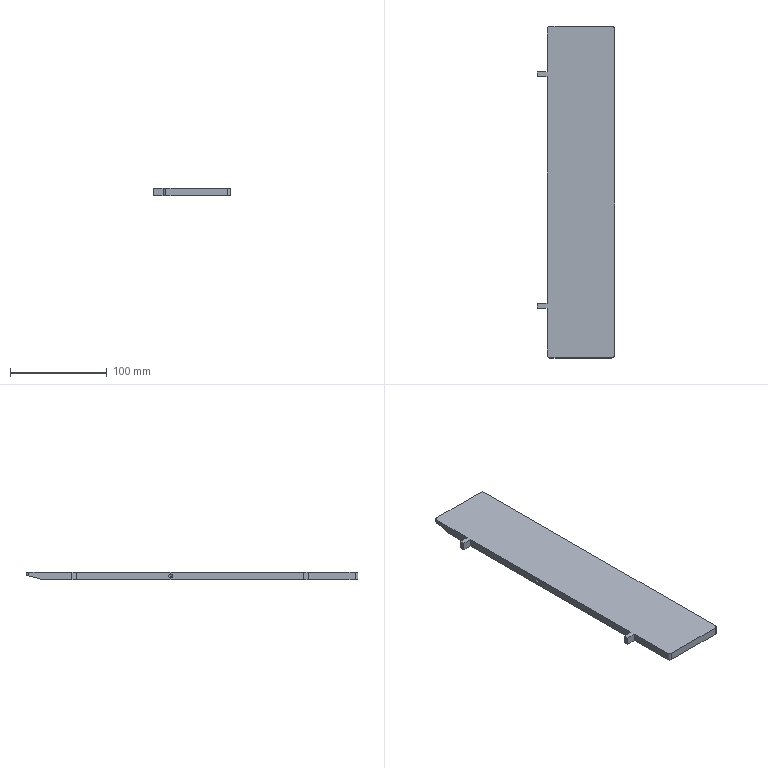Component | SolidWorks | SecondGenerationFour-sidedLabelingFeedingRearBaffle-1 | 1 solid | 23 faces | box 80 x 344 x 8 mm | volume 189871 mm3 | plane 15 | cylinder 6 | cone 2 | commonest cylinder face diameters 6 x4 4.2 x2
build123d program:
from build123d import *

# Parameters (mm, degrees)
SKETCH1_W             = 8
SKETCH1_H             = 345
BOSS_EXTRUDE1_DEPTH   = 70
M5_TAPPED_HOLE1_D     = 4.2
M5_TAPPED_HOLE1_DEPTH = 18.4
M5_TAPPED_HOLE1_TIP   = 1.262
SKETCH7_W             = 154.93
SKETCH7_H             = 42.695
CUT_EXTRUDE2_DEPTH    = 353.121
CHAMFER1_SIZE         = 5
CHAMFER1_SIZE2        = 18.66
FILLET1_R             = 3
SKETCH5_W             = 8
SKETCH5_H             = 5
BOSS_EXTRUDE2_DEPTH   = 10


with BuildPart() as part:
    # Sketch1 → Boss-Extrude1 (new body)
    with BuildSketch(Plane.XY):
        with Locations((-4, 172.5)):
            Rectangle(SKETCH1_W, SKETCH1_H)
    extrude(amount=BOSS_EXTRUDE1_DEPTH)

    # M5 Tapped Hole1
    with Locations(Plane(origin=(0, 0, 0), x_dir=(-1, 0, 0), z_dir=(0, 0, -1))):
        with Locations((4, 195)):
            Hole(M5_TAPPED_HOLE1_D / 2, depth=M5_TAPPED_HOLE1_DEPTH)
            with Locations((0, 0, -(M5_TAPPED_HOLE1_DEPTH + M5_TAPPED_HOLE1_TIP / 2))):  # 118° drill point
                Cone(0, M5_TAPPED_HOLE1_D / 2, M5_TAPPED_HOLE1_TIP, mode=Mode.SUBTRACT)

    # Sketch7 → Cut-Extrude2 (cut, through all)
    with BuildSketch(Plane.ZY.offset(8)):
        with Locations((38.651, -20.347)):
            Rectangle(SKETCH7_W, SKETCH7_H)
    extrude(amount=-CUT_EXTRUDE2_DEPTH, mode=Mode.SUBTRACT)

    # Chamfer1
    chamfer1_edges = [part.edges().sort_by_distance(p)[0] for p in [
        (0, 345, 35),
    ]]
    chamfer1_side = [part.faces().sort_by_distance(p)[0] for p in [
        (-4, 345, 35),
    ]]
    chamfer(chamfer1_edges, length=CHAMFER1_SIZE, length2=CHAMFER1_SIZE2, reference=chamfer1_side[0])

    # Fillet1
    fillet1_edges = [part.edges().sort_by_distance(p)[0] for p in [
        (-4, 1, 0),
        (-4, 1, 70),
        (-6.5, 345, 0),
        (-6.5, 345, 70),
    ]]
    fillet(fillet1_edges, radius=FILLET1_R)

    # Sketch5 → Boss-Extrude2 (add)
    with BuildSketch(Plane(origin=(0, 0, 0), x_dir=(-1, 0, 0), z_dir=(0, 0, -1))):
        with Locations((4, 295)):
            Rectangle(SKETCH5_W, SKETCH5_H)
        with Locations((4, 55)):
            Rectangle(SKETCH5_W, SKETCH5_H)
    extrude(amount=BOSS_EXTRUDE2_DEPTH)


solid = part.part

# Placed as in the assembly
solid = solid.moved(Location((-70.027, 46.863, -32), (0, 90, 0)))
STEP:
#1=CARTESIAN_POINT('',(-2.033,9.522,-1.185));
#2=VERTEX_POINT('',#1);
#3=CARTESIAN_POINT('',(-2.033,9.522,-1.02));
#4=VERTEX_POINT('',#3);
#5=CARTESIAN_POINT('',(-2.033,9.522,-1.102));
#6=DIRECTION('',(-1.,0.,0.));
#7=DIRECTION('',(0.,0.,1.));
#8=AXIS2_PLACEMENT_3D('',#5,#6,#7);
#9=CIRCLE('',#8,0.08268);
#10=EDGE_CURVE('',#2,#4,#9,.T.);
#11=ORIENTED_EDGE('',*,*,#10,.F.);
#12=CARTESIAN_POINT('',(-2.757,9.522,-1.185));
#13=VERTEX_POINT('',#12);
#14=CARTESIAN_POINT('',(-2.757,9.522,-1.185));
#15=DIRECTION('',(-1.,0.,0.));
#16=VECTOR('',#15,39.37);
#17=LINE('',#14,#16);
#18=EDGE_CURVE('',#2,#13,#17,.T.);
#19=ORIENTED_EDGE('',*,*,#18,.T.);
#20=CARTESIAN_POINT('',(-2.757,9.522,-1.02));
#21=VERTEX_POINT('',#20);
#22=CARTESIAN_POINT('',(-2.757,9.522,-1.102));
#23=DIRECTION('',(-1.,0.,0.));
#24=DIRECTION('',(0.,0.,1.));
#25=AXIS2_PLACEMENT_3D('',#22,#23,#24);
#26=CIRCLE('',#25,0.08268);
#27=EDGE_CURVE('',#13,#21,#26,.T.);
#28=ORIENTED_EDGE('',*,*,#27,.T.);
#29=CARTESIAN_POINT('',(-2.757,9.522,-1.02));
#30=DIRECTION('',(-1.,0.,0.));
#31=VECTOR('',#30,39.37);
#32=LINE('',#29,#31);
#33=EDGE_CURVE('',#4,#21,#32,.T.);
#34=ORIENTED_EDGE('',*,*,#33,.F.);
#35=EDGE_LOOP('',(#11,#19,#28,#34));
#36=FACE_OUTER_BOUND('',#35,.T.);
#37=CARTESIAN_POINT('',(-2.757,9.522,-1.102));
#38=DIRECTION('',(-1.,0.,0.));
#39=DIRECTION('',(0.,0.,1.));
#40=AXIS2_PLACEMENT_3D('',#37,#38,#39);
#41=CYLINDRICAL_SURFACE('',#40,0.08268);
#42=ADVANCED_FACE('',(#36),#41,.F.);
#43=CARTESIAN_POINT('',(-1.983,9.522,-1.102));
#44=VERTEX_POINT('',#43);
#45=CARTESIAN_POINT('',(-2.033,9.522,-1.02));
#46=DIRECTION('',(-0.515,-0.,0.8572));
#47=VECTOR('',#46,39.37);
#48=LINE('',#45,#47);
#49=EDGE_CURVE('',#44,#4,#48,.T.);
#50=ORIENTED_EDGE('',*,*,#49,.F.);
#51=CARTESIAN_POINT('',(-2.033,9.522,-1.185));
#52=DIRECTION('',(-0.515,0.,-0.8572));
#53=VECTOR('',#52,39.37);
#54=LINE('',#51,#53);
#55=EDGE_CURVE('',#44,#2,#54,.T.);
#56=ORIENTED_EDGE('',*,*,#55,.T.);
#57=ORIENTED_EDGE('',*,*,#10,.T.);
#58=EDGE_LOOP('',(#50,#56,#57));
#59=FACE_OUTER_BOUND('',#58,.T.);
#60=CARTESIAN_POINT('',(-2.033,9.522,-1.102));
#61=DIRECTION('',(-1.,0.,0.));
#62=DIRECTION('',(0.,0.,1.));
#63=AXIS2_PLACEMENT_3D('',#60,#61,#62);
#64=CONICAL_SURFACE('',#63,0.08268,1.03);
#65=ADVANCED_FACE('',(#59),#64,.F.);
#66=CARTESIAN_POINT('',(-2.757,9.522,-1.102));
#67=DIRECTION('',(-1.,0.,0.));
#68=DIRECTION('',(0.,0.,1.));
#69=AXIS2_PLACEMENT_3D('',#66,#67,#68);
#70=CIRCLE('',#69,0.08268);
#71=EDGE_CURVE('',#21,#13,#70,.T.);
#72=ORIENTED_EDGE('',*,*,#71,.F.);
#73=ORIENTED_EDGE('',*,*,#27,.F.);
#74=EDGE_LOOP('',(#72,#73));
#75=FACE_BOUND('',#74,.T.);
#76=CARTESIAN_POINT('',(-2.757,4.109,-1.26));
#77=VERTEX_POINT('',#76);
#78=CARTESIAN_POINT('',(-2.757,13.361,-1.26));
#79=VERTEX_POINT('',#78);
#80=CARTESIAN_POINT('',(-2.757,1.845,-1.26));
#81=DIRECTION('',(0.,1.,0.));
#82=VECTOR('',#81,39.37);
#83=LINE('',#80,#82);
#84=EDGE_CURVE('',#77,#79,#83,.T.);
#85=ORIENTED_EDGE('',*,*,#84,.F.);
#86=CARTESIAN_POINT('',(-2.757,4.109,-0.9449));
#87=VERTEX_POINT('',#86);
#88=CARTESIAN_POINT('',(-2.757,4.109,-0.9449));
#89=DIRECTION('',(0.,0.,-1.));
#90=VECTOR('',#89,39.37);
#91=LINE('',#88,#90);
#92=EDGE_CURVE('',#87,#77,#91,.T.);
#93=ORIENTED_EDGE('',*,*,#92,.F.);
#94=CARTESIAN_POINT('',(-2.757,13.361,-0.9449));
#95=VERTEX_POINT('',#94);
#96=CARTESIAN_POINT('',(-2.757,1.845,-0.9449));
#97=DIRECTION('',(0.,-1.,-0.));
#98=VECTOR('',#97,39.37);
#99=LINE('',#96,#98);
#100=EDGE_CURVE('',#95,#87,#99,.T.);
#101=ORIENTED_EDGE('',*,*,#100,.F.);
#102=CARTESIAN_POINT('',(-2.757,13.361,-1.26));
#103=DIRECTION('',(0.,-0.,1.));
#104=VECTOR('',#103,39.37);
#105=LINE('',#102,#104);
#106=EDGE_CURVE('',#79,#95,#105,.T.);
#107=ORIENTED_EDGE('',*,*,#106,.F.);
#108=EDGE_LOOP('',(#85,#93,#101,#107));
#109=FACE_OUTER_BOUND('',#108,.T.);
#110=CARTESIAN_POINT('',(-2.757,15.428,-0.9449));
#111=DIRECTION('',(-1.,0.,0.));
#112=DIRECTION('',(0.,-0.,1.));
#113=AXIS2_PLACEMENT_3D('',#110,#111,#112);
#114=PLANE('',#113);
#115=ADVANCED_FACE('',(#75,#109),#114,.T.);
#116=CARTESIAN_POINT('',(-2.757,3.912,-0.9449));
#117=VERTEX_POINT('',#116);
#118=CARTESIAN_POINT('',(-2.757,2.002,-0.9449));
#119=VERTEX_POINT('',#118);
#120=CARTESIAN_POINT('',(-2.757,1.845,-0.9449));
#121=DIRECTION('',(0.,-1.,-0.));
#122=VECTOR('',#121,39.37);
#123=LINE('',#120,#122);
#124=EDGE_CURVE('',#117,#119,#123,.T.);
#125=ORIENTED_EDGE('',*,*,#124,.F.);
#126=CARTESIAN_POINT('',(-2.757,3.912,-1.26));
#127=VERTEX_POINT('',#126);
#128=CARTESIAN_POINT('',(-2.757,3.912,-0.9449));
#129=DIRECTION('',(0.,-0.,1.));
#130=VECTOR('',#129,39.37);
#131=LINE('',#128,#130);
#132=EDGE_CURVE('',#127,#117,#131,.T.);
#133=ORIENTED_EDGE('',*,*,#132,.F.);
#134=CARTESIAN_POINT('',(-2.757,2.002,-1.26));
#135=VERTEX_POINT('',#134);
#136=CARTESIAN_POINT('',(-2.757,1.845,-1.26));
#137=DIRECTION('',(0.,1.,0.));
#138=VECTOR('',#137,39.37);
#139=LINE('',#136,#138);
#140=EDGE_CURVE('',#135,#127,#139,.T.);
#141=ORIENTED_EDGE('',*,*,#140,.F.);
#142=CARTESIAN_POINT('',(-2.757,2.002,-0.9449));
#143=DIRECTION('',(0.,-0.,1.));
#144=VECTOR('',#143,39.37);
#145=LINE('',#142,#144);
#146=EDGE_CURVE('',#135,#119,#145,.T.);
#147=ORIENTED_EDGE('',*,*,#146,.T.);
#148=EDGE_LOOP('',(#125,#133,#141,#147));
#149=FACE_OUTER_BOUND('',#148,.T.);
#150=CARTESIAN_POINT('',(-2.757,15.428,-0.9449));
#151=DIRECTION('',(-1.,0.,0.));
#152=DIRECTION('',(0.,-0.,1.));
#153=AXIS2_PLACEMENT_3D('',#150,#151,#152);
#154=PLANE('',#153);
#155=ADVANCED_FACE('',(#149),#154,.T.);
#156=CARTESIAN_POINT('',(-2.757,13.558,-1.26));
#157=VERTEX_POINT('',#156);
#158=CARTESIAN_POINT('',(-2.757,14.693,-1.26));
#159=VERTEX_POINT('',#158);
#160=CARTESIAN_POINT('',(-2.757,1.845,-1.26));
#161=DIRECTION('',(0.,1.,0.));
#162=VECTOR('',#161,39.37);
#163=LINE('',#160,#162);
#164=EDGE_CURVE('',#157,#159,#163,.T.);
#165=ORIENTED_EDGE('',*,*,#164,.F.);
#166=CARTESIAN_POINT('',(-2.757,13.558,-0.9449));
#167=VERTEX_POINT('',#166);
#168=CARTESIAN_POINT('',(-2.757,13.558,-1.26));
#169=DIRECTION('',(0.,0.,-1.));
#170=VECTOR('',#169,39.37);
#171=LINE('',#168,#170);
#172=EDGE_CURVE('',#167,#157,#171,.T.);
#173=ORIENTED_EDGE('',*,*,#172,.F.);
#174=CARTESIAN_POINT('',(-2.757,15.31,-0.9449));
#175=VERTEX_POINT('',#174);
#176=CARTESIAN_POINT('',(-2.757,1.845,-0.9449));
#177=DIRECTION('',(0.,-1.,-0.));
#178=VECTOR('',#177,39.37);
#179=LINE('',#176,#178);
#180=EDGE_CURVE('',#175,#167,#179,.T.);
#181=ORIENTED_EDGE('',*,*,#180,.F.);
#182=CARTESIAN_POINT('',(-2.757,15.31,-1.095));
#183=VERTEX_POINT('',#182);
#184=CARTESIAN_POINT('',(-2.757,15.31,-1.063));
#185=DIRECTION('',(0.,0.,-1.));
#186=VECTOR('',#185,39.37);
#187=LINE('',#184,#186);
#188=EDGE_CURVE('',#175,#183,#187,.T.);
#189=ORIENTED_EDGE('',*,*,#188,.T.);
#190=CARTESIAN_POINT('',(-2.757,15.457,-1.055));
#191=DIRECTION('',(0.,-0.9659,-0.2588));
#192=VECTOR('',#191,39.37);
#193=LINE('',#190,#192);
#194=EDGE_CURVE('',#183,#159,#193,.T.);
#195=ORIENTED_EDGE('',*,*,#194,.T.);
#196=EDGE_LOOP('',(#165,#173,#181,#189,#195));
#197=FACE_OUTER_BOUND('',#196,.T.);
#198=CARTESIAN_POINT('',(-2.757,15.428,-0.9449));
#199=DIRECTION('',(-1.,0.,0.));
#200=DIRECTION('',(0.,-0.,1.));
#201=AXIS2_PLACEMENT_3D('',#198,#199,#200);
#202=PLANE('',#201);
#203=ADVANCED_FACE('',(#197),#202,.T.);
#204=CARTESIAN_POINT('',(-0.1192,1.884,-0.9449));
#205=VERTEX_POINT('',#204);
#206=CARTESIAN_POINT('',(-2.639,1.884,-0.9449));
#207=VERTEX_POINT('',#206);
#208=CARTESIAN_POINT('',(-4.285,1.884,-0.9449));
#209=DIRECTION('',(-1.,0.,0.));
#210=VECTOR('',#209,39.37);
#211=LINE('',#208,#210);
#212=EDGE_CURVE('',#205,#207,#211,.T.);
#213=ORIENTED_EDGE('',*,*,#212,.F.);
#214=CARTESIAN_POINT('',(-0.001059,2.002,-0.9449));
#215=VERTEX_POINT('',#214);
#216=CARTESIAN_POINT('',(-0.1192,2.002,-0.9449));
#217=DIRECTION('',(0.,-0.,1.));
#218=DIRECTION('',(-1.,0.,0.));
#219=AXIS2_PLACEMENT_3D('',#216,#217,#218);
#220=CIRCLE('',#219,0.1181);
#221=EDGE_CURVE('',#205,#215,#220,.T.);
#222=ORIENTED_EDGE('',*,*,#221,.T.);
#223=CARTESIAN_POINT('',(-0.001059,15.31,-0.9449));
#224=VERTEX_POINT('',#223);
#225=CARTESIAN_POINT('',(-0.001059,1.845,-0.9449));
#226=DIRECTION('',(0.,-1.,-0.));
#227=VECTOR('',#226,39.37);
#228=LINE('',#225,#227);
#229=EDGE_CURVE('',#224,#215,#228,.T.);
#230=ORIENTED_EDGE('',*,*,#229,.F.);
#231=CARTESIAN_POINT('',(-0.1192,15.428,-0.9449));
#232=VERTEX_POINT('',#231);
#233=CARTESIAN_POINT('',(-0.1192,15.31,-0.9449));
#234=DIRECTION('',(0.,-0.,1.));
#235=DIRECTION('',(-1.,0.,0.));
#236=AXIS2_PLACEMENT_3D('',#233,#234,#235);
#237=CIRCLE('',#236,0.1181);
#238=EDGE_CURVE('',#224,#232,#237,.T.);
#239=ORIENTED_EDGE('',*,*,#238,.T.);
#240=CARTESIAN_POINT('',(-2.639,15.428,-0.9449));
#241=VERTEX_POINT('',#240);
#242=CARTESIAN_POINT('',(-0.001059,15.428,-0.9449));
#243=DIRECTION('',(-1.,0.,0.));
#244=VECTOR('',#243,39.37);
#245=LINE('',#242,#244);
#246=EDGE_CURVE('',#232,#241,#245,.T.);
#247=ORIENTED_EDGE('',*,*,#246,.T.);
#248=CARTESIAN_POINT('',(-2.639,15.31,-0.9449));
#249=DIRECTION('',(0.,-0.,1.));
#250=DIRECTION('',(-1.,0.,0.));
#251=AXIS2_PLACEMENT_3D('',#248,#249,#250);
#252=CIRCLE('',#251,0.1181);
#253=EDGE_CURVE('',#241,#175,#252,.T.);
#254=ORIENTED_EDGE('',*,*,#253,.T.);
#255=ORIENTED_EDGE('',*,*,#180,.T.);
#256=CARTESIAN_POINT('',(-3.151,13.558,-0.9449));
#257=VERTEX_POINT('',#256);
#258=CARTESIAN_POINT('',(-3.151,13.558,-0.9449));
#259=DIRECTION('',(1.,0.,0.));
#260=VECTOR('',#259,39.37);
#261=LINE('',#258,#260);
#262=EDGE_CURVE('',#257,#167,#261,.T.);
#263=ORIENTED_EDGE('',*,*,#262,.F.);
#264=CARTESIAN_POINT('',(-3.151,13.361,-0.9449));
#265=VERTEX_POINT('',#264);
#266=CARTESIAN_POINT('',(-3.151,13.558,-0.9449));
#267=DIRECTION('',(0.,1.,0.));
#268=VECTOR('',#267,39.37);
#269=LINE('',#266,#268);
#270=EDGE_CURVE('',#265,#257,#269,.T.);
#271=ORIENTED_EDGE('',*,*,#270,.F.);
#272=CARTESIAN_POINT('',(-3.151,13.361,-0.9449));
#273=DIRECTION('',(1.,0.,0.));
#274=VECTOR('',#273,39.37);
#275=LINE('',#272,#274);
#276=EDGE_CURVE('',#265,#95,#275,.T.);
#277=ORIENTED_EDGE('',*,*,#276,.T.);
#278=ORIENTED_EDGE('',*,*,#100,.T.);
#279=CARTESIAN_POINT('',(-3.151,4.109,-0.9449));
#280=VERTEX_POINT('',#279);
#281=CARTESIAN_POINT('',(-3.151,4.109,-0.9449));
#282=DIRECTION('',(1.,0.,0.));
#283=VECTOR('',#282,39.37);
#284=LINE('',#281,#283);
#285=EDGE_CURVE('',#280,#87,#284,.T.);
#286=ORIENTED_EDGE('',*,*,#285,.F.);
#287=CARTESIAN_POINT('',(-3.151,3.912,-0.9449));
#288=VERTEX_POINT('',#287);
#289=CARTESIAN_POINT('',(-3.151,4.109,-0.9449));
#290=DIRECTION('',(0.,1.,0.));
#291=VECTOR('',#290,39.37);
#292=LINE('',#289,#291);
#293=EDGE_CURVE('',#288,#280,#292,.T.);
#294=ORIENTED_EDGE('',*,*,#293,.F.);
#295=CARTESIAN_POINT('',(-3.151,3.912,-0.9449));
#296=DIRECTION('',(1.,0.,0.));
#297=VECTOR('',#296,39.37);
#298=LINE('',#295,#297);
#299=EDGE_CURVE('',#288,#117,#298,.T.);
#300=ORIENTED_EDGE('',*,*,#299,.T.);
#301=ORIENTED_EDGE('',*,*,#124,.T.);
#302=CARTESIAN_POINT('',(-2.639,2.002,-0.9449));
#303=DIRECTION('',(0.,-0.,1.));
#304=DIRECTION('',(-1.,0.,0.));
#305=AXIS2_PLACEMENT_3D('',#302,#303,#304);
#306=CIRCLE('',#305,0.1181);
#307=EDGE_CURVE('',#119,#207,#306,.T.);
#308=ORIENTED_EDGE('',*,*,#307,.T.);
#309=EDGE_LOOP('',(#213,#222,#230,#239,#247,#254,#255,#263,#271,#277,#278,#286,#294,#300,#301,#308));
#310=FACE_OUTER_BOUND('',#309,.T.);
#311=CARTESIAN_POINT('',(-0.001059,1.845,-0.9449));
#312=DIRECTION('',(0.,0.,-1.));
#313=DIRECTION('',(-1.,0.,0.));
#314=AXIS2_PLACEMENT_3D('',#311,#312,#313);
#315=PLANE('',#314);
#316=ADVANCED_FACE('',(#310),#315,.F.);
#317=CARTESIAN_POINT('',(-0.001059,2.002,-1.26));
#318=VERTEX_POINT('',#317);
#319=CARTESIAN_POINT('',(-0.001059,14.693,-1.26));
#320=VERTEX_POINT('',#319);
#321=CARTESIAN_POINT('',(-0.001059,1.845,-1.26));
#322=DIRECTION('',(0.,1.,0.));
#323=VECTOR('',#322,39.37);
#324=LINE('',#321,#323);
#325=EDGE_CURVE('',#318,#320,#324,.T.);
#326=ORIENTED_EDGE('',*,*,#325,.F.);
#327=CARTESIAN_POINT('',(-0.1192,1.884,-1.26));
#328=VERTEX_POINT('',#327);
#329=CARTESIAN_POINT('',(-0.1192,2.002,-1.26));
#330=DIRECTION('',(0.,0.,-1.));
#331=DIRECTION('',(1.,0.,0.));
#332=AXIS2_PLACEMENT_3D('',#329,#330,#331);
#333=CIRCLE('',#332,0.1181);
#334=EDGE_CURVE('',#318,#328,#333,.T.);
#335=ORIENTED_EDGE('',*,*,#334,.T.);
#336=CARTESIAN_POINT('',(-2.639,1.884,-1.26));
#337=VERTEX_POINT('',#336);
#338=CARTESIAN_POINT('',(-4.285,1.884,-1.26));
#339=DIRECTION('',(-1.,0.,0.));
#340=VECTOR('',#339,39.37);
#341=LINE('',#338,#340);
#342=EDGE_CURVE('',#328,#337,#341,.T.);
#343=ORIENTED_EDGE('',*,*,#342,.T.);
#344=CARTESIAN_POINT('',(-2.639,2.002,-1.26));
#345=DIRECTION('',(0.,0.,-1.));
#346=DIRECTION('',(1.,0.,0.));
#347=AXIS2_PLACEMENT_3D('',#344,#345,#346);
#348=CIRCLE('',#347,0.1181);
#349=EDGE_CURVE('',#337,#135,#348,.T.);
#350=ORIENTED_EDGE('',*,*,#349,.T.);
#351=ORIENTED_EDGE('',*,*,#140,.T.);
#352=CARTESIAN_POINT('',(-3.151,3.912,-1.26));
#353=VERTEX_POINT('',#352);
#354=CARTESIAN_POINT('',(-3.151,3.912,-1.26));
#355=DIRECTION('',(1.,0.,0.));
#356=VECTOR('',#355,39.37);
#357=LINE('',#354,#356);
#358=EDGE_CURVE('',#353,#127,#357,.T.);
#359=ORIENTED_EDGE('',*,*,#358,.F.);
#360=CARTESIAN_POINT('',(-3.151,4.109,-1.26));
#361=VERTEX_POINT('',#360);
#362=CARTESIAN_POINT('',(-3.151,4.109,-1.26));
#363=DIRECTION('',(0.,-1.,-0.));
#364=VECTOR('',#363,39.37);
#365=LINE('',#362,#364);
#366=EDGE_CURVE('',#361,#353,#365,.T.);
#367=ORIENTED_EDGE('',*,*,#366,.F.);
#368=CARTESIAN_POINT('',(-3.151,4.109,-1.26));
#369=DIRECTION('',(1.,0.,0.));
#370=VECTOR('',#369,39.37);
#371=LINE('',#368,#370);
#372=EDGE_CURVE('',#361,#77,#371,.T.);
#373=ORIENTED_EDGE('',*,*,#372,.T.);
#374=ORIENTED_EDGE('',*,*,#84,.T.);
#375=CARTESIAN_POINT('',(-3.151,13.361,-1.26));
#376=VERTEX_POINT('',#375);
#377=CARTESIAN_POINT('',(-3.151,13.361,-1.26));
#378=DIRECTION('',(1.,0.,0.));
#379=VECTOR('',#378,39.37);
#380=LINE('',#377,#379);
#381=EDGE_CURVE('',#376,#79,#380,.T.);
#382=ORIENTED_EDGE('',*,*,#381,.F.);
#383=CARTESIAN_POINT('',(-3.151,13.558,-1.26));
#384=VERTEX_POINT('',#383);
#385=CARTESIAN_POINT('',(-3.151,13.558,-1.26));
#386=DIRECTION('',(0.,-1.,-0.));
#387=VECTOR('',#386,39.37);
#388=LINE('',#385,#387);
#389=EDGE_CURVE('',#384,#376,#388,.T.);
#390=ORIENTED_EDGE('',*,*,#389,.F.);
#391=CARTESIAN_POINT('',(-3.151,13.558,-1.26));
#392=DIRECTION('',(1.,0.,0.));
#393=VECTOR('',#392,39.37);
#394=LINE('',#391,#393);
#395=EDGE_CURVE('',#384,#157,#394,.T.);
#396=ORIENTED_EDGE('',*,*,#395,.T.);
#397=ORIENTED_EDGE('',*,*,#164,.T.);
#398=CARTESIAN_POINT('',(-0.001059,14.693,-1.26));
#399=DIRECTION('',(1.,0.,0.));
#400=VECTOR('',#399,39.37);
#401=LINE('',#398,#400);
#402=EDGE_CURVE('',#159,#320,#401,.T.);
#403=ORIENTED_EDGE('',*,*,#402,.T.);
#404=EDGE_LOOP('',(#326,#335,#343,#350,#351,#359,#367,#373,#374,#382,#390,#396,#397,#403));
#405=FACE_OUTER_BOUND('',#404,.T.);
#406=CARTESIAN_POINT('',(-0.001059,1.845,-1.26));
#407=DIRECTION('',(0.,-0.,1.));
#408=DIRECTION('',(1.,0.,0.));
#409=AXIS2_PLACEMENT_3D('',#406,#407,#408);
#410=PLANE('',#409);
#411=ADVANCED_FACE('',(#405),#410,.F.);
#412=ORIENTED_EDGE('',*,*,#246,.F.);
#413=CARTESIAN_POINT('',(-0.1192,15.428,-1.063));
#414=VERTEX_POINT('',#413);
#415=CARTESIAN_POINT('',(-0.1192,15.428,-0.9449));
#416=DIRECTION('',(0.,0.,-1.));
#417=VECTOR('',#416,39.37);
#418=LINE('',#415,#417);
#419=EDGE_CURVE('',#232,#414,#418,.T.);
#420=ORIENTED_EDGE('',*,*,#419,.T.);
#421=CARTESIAN_POINT('',(-2.639,15.428,-1.063));
#422=VERTEX_POINT('',#421);
#423=CARTESIAN_POINT('',(-0.001059,15.428,-1.063));
#424=DIRECTION('',(-1.,0.,0.));
#425=VECTOR('',#424,39.37);
#426=LINE('',#423,#425);
#427=EDGE_CURVE('',#414,#422,#426,.T.);
#428=ORIENTED_EDGE('',*,*,#427,.T.);
#429=CARTESIAN_POINT('',(-2.639,15.428,-0.9449));
#430=DIRECTION('',(0.,-0.,1.));
#431=VECTOR('',#430,39.37);
#432=LINE('',#429,#431);
#433=EDGE_CURVE('',#422,#241,#432,.T.);
#434=ORIENTED_EDGE('',*,*,#433,.T.);
#435=EDGE_LOOP('',(#412,#420,#428,#434));
#436=FACE_OUTER_BOUND('',#435,.T.);
#437=CARTESIAN_POINT('',(-0.001059,15.428,-0.9449));
#438=DIRECTION('',(0.,-1.,-0.));
#439=DIRECTION('',(-1.,0.,0.));
#440=AXIS2_PLACEMENT_3D('',#437,#438,#439);
#441=PLANE('',#440);
#442=ADVANCED_FACE('',(#436),#441,.F.);
#443=ORIENTED_EDGE('',*,*,#229,.T.);
#444=CARTESIAN_POINT('',(-0.001059,2.002,-0.9449));
#445=DIRECTION('',(0.,0.,-1.));
#446=VECTOR('',#445,39.37);
#447=LINE('',#444,#446);
#448=EDGE_CURVE('',#215,#318,#447,.T.);
#449=ORIENTED_EDGE('',*,*,#448,.T.);
#450=ORIENTED_EDGE('',*,*,#325,.T.);
#451=CARTESIAN_POINT('',(-0.001059,15.31,-1.095));
#452=VERTEX_POINT('',#451);
#453=CARTESIAN_POINT('',(-0.001059,15.428,-1.063));
#454=DIRECTION('',(0.,0.9659,0.2588));
#455=VECTOR('',#454,39.37);
#456=LINE('',#453,#455);
#457=EDGE_CURVE('',#320,#452,#456,.T.);
#458=ORIENTED_EDGE('',*,*,#457,.T.);
#459=CARTESIAN_POINT('',(-0.001059,15.31,-0.9449));
#460=DIRECTION('',(0.,-0.,1.));
#461=VECTOR('',#460,39.37);
#462=LINE('',#459,#461);
#463=EDGE_CURVE('',#452,#224,#462,.T.);
#464=ORIENTED_EDGE('',*,*,#463,.T.);
#465=EDGE_LOOP('',(#443,#449,#450,#458,#464));
#466=FACE_OUTER_BOUND('',#465,.T.);
#467=CARTESIAN_POINT('',(-0.001059,15.428,-0.9449));
#468=DIRECTION('',(-1.,0.,0.));
#469=DIRECTION('',(0.,-0.,1.));
#470=AXIS2_PLACEMENT_3D('',#467,#468,#469);
#471=PLANE('',#470);
#472=ADVANCED_FACE('',(#466),#471,.F.);
#473=ORIENTED_EDGE('',*,*,#55,.F.);
#474=ORIENTED_EDGE('',*,*,#49,.T.);
#475=CARTESIAN_POINT('',(-2.033,9.522,-1.102));
#476=DIRECTION('',(-1.,0.,0.));
#477=DIRECTION('',(0.,0.,1.));
#478=AXIS2_PLACEMENT_3D('',#475,#476,#477);
#479=CIRCLE('',#478,0.08268);
#480=EDGE_CURVE('',#4,#2,#479,.T.);
#481=ORIENTED_EDGE('',*,*,#480,.T.);
#482=EDGE_LOOP('',(#473,#474,#481));
#483=FACE_OUTER_BOUND('',#482,.T.);
#484=CARTESIAN_POINT('',(-2.033,9.522,-1.102));
#485=DIRECTION('',(-1.,0.,0.));
#486=DIRECTION('',(0.,0.,1.));
#487=AXIS2_PLACEMENT_3D('',#484,#485,#486);
#488=CONICAL_SURFACE('',#487,0.08268,1.03);
#489=ADVANCED_FACE('',(#483),#488,.F.);
#490=ORIENTED_EDGE('',*,*,#18,.F.);
#491=ORIENTED_EDGE('',*,*,#480,.F.);
#492=ORIENTED_EDGE('',*,*,#33,.T.);
#493=ORIENTED_EDGE('',*,*,#71,.T.);
#494=EDGE_LOOP('',(#490,#491,#492,#493));
#495=FACE_OUTER_BOUND('',#494,.T.);
#496=CARTESIAN_POINT('',(-2.757,9.522,-1.102));
#497=DIRECTION('',(-1.,0.,0.));
#498=DIRECTION('',(0.,0.,1.));
#499=AXIS2_PLACEMENT_3D('',#496,#497,#498);
#500=CYLINDRICAL_SURFACE('',#499,0.08268);
#501=ADVANCED_FACE('',(#495),#500,.F.);
#502=ORIENTED_EDGE('',*,*,#342,.F.);
#503=CARTESIAN_POINT('',(-0.1192,1.884,-1.26));
#504=DIRECTION('',(0.,-0.,1.));
#505=VECTOR('',#504,39.37);
#506=LINE('',#503,#505);
#507=EDGE_CURVE('',#328,#205,#506,.T.);
#508=ORIENTED_EDGE('',*,*,#507,.T.);
#509=ORIENTED_EDGE('',*,*,#212,.T.);
#510=CARTESIAN_POINT('',(-2.639,1.884,-1.26));
#511=DIRECTION('',(0.,0.,-1.));
#512=VECTOR('',#511,39.37);
#513=LINE('',#510,#512);
#514=EDGE_CURVE('',#207,#337,#513,.T.);
#515=ORIENTED_EDGE('',*,*,#514,.T.);
#516=EDGE_LOOP('',(#502,#508,#509,#515));
#517=FACE_OUTER_BOUND('',#516,.T.);
#518=CARTESIAN_POINT('',(-4.285,1.884,-1.26));
#519=DIRECTION('',(0.,1.,0.));
#520=DIRECTION('',(0.,-0.,1.));
#521=AXIS2_PLACEMENT_3D('',#518,#519,#520);
#522=PLANE('',#521);
#523=ADVANCED_FACE('',(#517),#522,.F.);
#524=ORIENTED_EDGE('',*,*,#427,.F.);
#525=CARTESIAN_POINT('',(-0.1192,15.428,-1.063));
#526=CARTESIAN_POINT('',(-0.04998,15.428,-1.063));
#527=CARTESIAN_POINT('',(-0.001059,15.379,-1.076));
#528=CARTESIAN_POINT('',(-0.001059,15.31,-1.095));
#529=(BOUNDED_CURVE()B_SPLINE_CURVE(3,(#525,#526,#527,#528),.UNSPECIFIED.,.F.,.F.)B_SPLINE_CURVE_WITH_KNOTS((4,4),(0.,1.571),.UNSPECIFIED.)CURVE()GEOMETRIC_REPRESENTATION_ITEM()RATIONAL_B_SPLINE_CURVE((1.,0.8047,0.8047,1.))REPRESENTATION_ITEM(''));
#530=EDGE_CURVE('',#414,#452,#529,.T.);
#531=ORIENTED_EDGE('',*,*,#530,.T.);
#532=ORIENTED_EDGE('',*,*,#457,.F.);
#533=ORIENTED_EDGE('',*,*,#402,.F.);
#534=ORIENTED_EDGE('',*,*,#194,.F.);
#535=CARTESIAN_POINT('',(-2.757,15.31,-1.095));
#536=CARTESIAN_POINT('',(-2.757,15.379,-1.076));
#537=CARTESIAN_POINT('',(-2.708,15.428,-1.063));
#538=CARTESIAN_POINT('',(-2.639,15.428,-1.063));
#539=(BOUNDED_CURVE()B_SPLINE_CURVE(3,(#535,#536,#537,#538),.UNSPECIFIED.,.F.,.F.)B_SPLINE_CURVE_WITH_KNOTS((4,4),(1.571,3.142),.UNSPECIFIED.)CURVE()GEOMETRIC_REPRESENTATION_ITEM()RATIONAL_B_SPLINE_CURVE((1.,0.8047,0.8047,1.))REPRESENTATION_ITEM(''));
#540=EDGE_CURVE('',#183,#422,#539,.T.);
#541=ORIENTED_EDGE('',*,*,#540,.T.);
#542=EDGE_LOOP('',(#524,#531,#532,#533,#534,#541));
#543=FACE_OUTER_BOUND('',#542,.T.);
#544=CARTESIAN_POINT('',(-0.001059,15.428,-1.063));
#545=DIRECTION('',(0.,-0.2588,0.9659));
#546=DIRECTION('',(0.,-0.9659,-0.2588));
#547=AXIS2_PLACEMENT_3D('',#544,#545,#546);
#548=PLANE('',#547);
#549=ADVANCED_FACE('',(#543),#548,.F.);
#550=ORIENTED_EDGE('',*,*,#221,.F.);
#551=ORIENTED_EDGE('',*,*,#507,.F.);
#552=ORIENTED_EDGE('',*,*,#334,.F.);
#553=ORIENTED_EDGE('',*,*,#448,.F.);
#554=EDGE_LOOP('',(#550,#551,#552,#553));
#555=FACE_OUTER_BOUND('',#554,.T.);
#556=CARTESIAN_POINT('',(-0.1192,2.002,-0.9449));
#557=DIRECTION('',(0.,0.,-1.));
#558=DIRECTION('',(0.,1.,0.));
#559=AXIS2_PLACEMENT_3D('',#556,#557,#558);
#560=CYLINDRICAL_SURFACE('',#559,0.1181);
#561=ADVANCED_FACE('',(#555),#560,.T.);
#562=ORIENTED_EDGE('',*,*,#307,.F.);
#563=ORIENTED_EDGE('',*,*,#146,.F.);
#564=ORIENTED_EDGE('',*,*,#349,.F.);
#565=ORIENTED_EDGE('',*,*,#514,.F.);
#566=EDGE_LOOP('',(#562,#563,#564,#565));
#567=FACE_OUTER_BOUND('',#566,.T.);
#568=CARTESIAN_POINT('',(-2.639,2.002,-1.26));
#569=DIRECTION('',(0.,-0.,1.));
#570=DIRECTION('',(0.,-1.,0.));
#571=AXIS2_PLACEMENT_3D('',#568,#569,#570);
#572=CYLINDRICAL_SURFACE('',#571,0.1181);
#573=ADVANCED_FACE('',(#567),#572,.T.);
#574=ORIENTED_EDGE('',*,*,#530,.F.);
#575=ORIENTED_EDGE('',*,*,#419,.F.);
#576=ORIENTED_EDGE('',*,*,#238,.F.);
#577=ORIENTED_EDGE('',*,*,#463,.F.);
#578=EDGE_LOOP('',(#574,#575,#576,#577));
#579=FACE_OUTER_BOUND('',#578,.T.);
#580=CARTESIAN_POINT('',(-0.1192,15.31,-0.9449));
#581=DIRECTION('',(0.,-0.,1.));
#582=DIRECTION('',(1.,0.,0.));
#583=AXIS2_PLACEMENT_3D('',#580,#581,#582);
#584=CYLINDRICAL_SURFACE('',#583,0.1181);
#585=ADVANCED_FACE('',(#579),#584,.T.);
#586=ORIENTED_EDGE('',*,*,#540,.F.);
#587=ORIENTED_EDGE('',*,*,#188,.F.);
#588=ORIENTED_EDGE('',*,*,#253,.F.);
#589=ORIENTED_EDGE('',*,*,#433,.F.);
#590=EDGE_LOOP('',(#586,#587,#588,#589));
#591=FACE_OUTER_BOUND('',#590,.T.);
#592=CARTESIAN_POINT('',(-2.639,15.31,-0.9449));
#593=DIRECTION('',(0.,0.,-1.));
#594=DIRECTION('',(-1.,0.,0.));
#595=AXIS2_PLACEMENT_3D('',#592,#593,#594);
#596=CYLINDRICAL_SURFACE('',#595,0.1181);
#597=ADVANCED_FACE('',(#591),#596,.T.);
#598=ORIENTED_EDGE('',*,*,#106,.T.);
#599=ORIENTED_EDGE('',*,*,#276,.F.);
#600=CARTESIAN_POINT('',(-3.151,13.361,-1.26));
#601=DIRECTION('',(0.,-0.,1.));
#602=VECTOR('',#601,39.37);
#603=LINE('',#600,#602);
#604=EDGE_CURVE('',#376,#265,#603,.T.);
#605=ORIENTED_EDGE('',*,*,#604,.F.);
#606=ORIENTED_EDGE('',*,*,#381,.T.);
#607=EDGE_LOOP('',(#598,#599,#605,#606));
#608=FACE_OUTER_BOUND('',#607,.T.);
#609=CARTESIAN_POINT('',(-3.151,13.361,-1.26));
#610=DIRECTION('',(0.,1.,0.));
#611=DIRECTION('',(1.,0.,0.));
#612=AXIS2_PLACEMENT_3D('',#609,#610,#611);
#613=PLANE('',#612);
#614=ADVANCED_FACE('',(#608),#613,.F.);
#615=ORIENTED_EDGE('',*,*,#172,.T.);
#616=ORIENTED_EDGE('',*,*,#395,.F.);
#617=CARTESIAN_POINT('',(-3.151,13.558,-1.26));
#618=DIRECTION('',(0.,0.,-1.));
#619=VECTOR('',#618,39.37);
#620=LINE('',#617,#619);
#621=EDGE_CURVE('',#257,#384,#620,.T.);
#622=ORIENTED_EDGE('',*,*,#621,.F.);
#623=ORIENTED_EDGE('',*,*,#262,.T.);
#624=EDGE_LOOP('',(#615,#616,#622,#623));
#625=FACE_OUTER_BOUND('',#624,.T.);
#626=CARTESIAN_POINT('',(-3.151,13.558,-1.26));
#627=DIRECTION('',(0.,-1.,-0.));
#628=DIRECTION('',(-1.,0.,0.));
#629=AXIS2_PLACEMENT_3D('',#626,#627,#628);
#630=PLANE('',#629);
#631=ADVANCED_FACE('',(#625),#630,.F.);
#632=ORIENTED_EDGE('',*,*,#389,.T.);
#633=ORIENTED_EDGE('',*,*,#604,.T.);
#634=ORIENTED_EDGE('',*,*,#270,.T.);
#635=ORIENTED_EDGE('',*,*,#621,.T.);
#636=EDGE_LOOP('',(#632,#633,#634,#635));
#637=FACE_OUTER_BOUND('',#636,.T.);
#638=CARTESIAN_POINT('',(-3.151,13.361,-1.26));
#639=DIRECTION('',(-1.,0.,0.));
#640=DIRECTION('',(0.,-0.,1.));
#641=AXIS2_PLACEMENT_3D('',#638,#639,#640);
#642=PLANE('',#641);
#643=ADVANCED_FACE('',(#637),#642,.T.);
#644=ORIENTED_EDGE('',*,*,#92,.T.);
#645=ORIENTED_EDGE('',*,*,#372,.F.);
#646=CARTESIAN_POINT('',(-3.151,4.109,-0.9449));
#647=DIRECTION('',(0.,0.,-1.));
#648=VECTOR('',#647,39.37);
#649=LINE('',#646,#648);
#650=EDGE_CURVE('',#280,#361,#649,.T.);
#651=ORIENTED_EDGE('',*,*,#650,.F.);
#652=ORIENTED_EDGE('',*,*,#285,.T.);
#653=EDGE_LOOP('',(#644,#645,#651,#652));
#654=FACE_OUTER_BOUND('',#653,.T.);
#655=CARTESIAN_POINT('',(-3.151,4.109,-0.9449));
#656=DIRECTION('',(0.,-1.,-0.));
#657=DIRECTION('',(-1.,0.,0.));
#658=AXIS2_PLACEMENT_3D('',#655,#656,#657);
#659=PLANE('',#658);
#660=ADVANCED_FACE('',(#654),#659,.F.);
#661=ORIENTED_EDGE('',*,*,#132,.T.);
#662=ORIENTED_EDGE('',*,*,#299,.F.);
#663=CARTESIAN_POINT('',(-3.151,3.912,-0.9449));
#664=DIRECTION('',(0.,-0.,1.));
#665=VECTOR('',#664,39.37);
#666=LINE('',#663,#665);
#667=EDGE_CURVE('',#353,#288,#666,.T.);
#668=ORIENTED_EDGE('',*,*,#667,.F.);
#669=ORIENTED_EDGE('',*,*,#358,.T.);
#670=EDGE_LOOP('',(#661,#662,#668,#669));
#671=FACE_OUTER_BOUND('',#670,.T.);
#672=CARTESIAN_POINT('',(-3.151,3.912,-0.9449));
#673=DIRECTION('',(0.,1.,0.));
#674=DIRECTION('',(1.,0.,0.));
#675=AXIS2_PLACEMENT_3D('',#672,#673,#674);
#676=PLANE('',#675);
#677=ADVANCED_FACE('',(#671),#676,.F.);
#678=ORIENTED_EDGE('',*,*,#293,.T.);
#679=ORIENTED_EDGE('',*,*,#650,.T.);
#680=ORIENTED_EDGE('',*,*,#366,.T.);
#681=ORIENTED_EDGE('',*,*,#667,.T.);
#682=EDGE_LOOP('',(#678,#679,#680,#681));
#683=FACE_OUTER_BOUND('',#682,.T.);
#684=CARTESIAN_POINT('',(-3.151,3.912,-0.9449));
#685=DIRECTION('',(1.,0.,0.));
#686=DIRECTION('',(0.,0.,-1.));
#687=AXIS2_PLACEMENT_3D('',#684,#685,#686);
#688=PLANE('',#687);
#689=ADVANCED_FACE('',(#683),#688,.F.);
#690=CLOSED_SHELL('',(#42,#65,#115,#155,#203,#316,#411,#442,#472,#489,#501,#523,#549,#561,#573,#585,#597,#614,#631,#643,#660,#677,#689));
#691=MANIFOLD_SOLID_BREP('',#690);
#692=CARTESIAN_POINT('',(0.,0.,0.));
#693=DIRECTION('',(0.,0.,1.));
#694=DIRECTION('',(1.,0.,0.));
#695=AXIS2_PLACEMENT_3D('',#692,#693,#694);
#696=(LENGTH_UNIT()NAMED_UNIT(*)SI_UNIT($,.METRE.));
#697=LENGTH_MEASURE_WITH_UNIT(LENGTH_MEASURE(0.0254),#696);
#698=DIMENSIONAL_EXPONENTS(1.,0.,0.,0.,0.,0.,0.);
#699=(CONVERSION_BASED_UNIT('',#697)LENGTH_UNIT()NAMED_UNIT(#698));
#700=UNCERTAINTY_MEASURE_WITH_UNIT(LENGTH_MEASURE(0.00001),#699,'','');
#701=(NAMED_UNIT(*)PLANE_ANGLE_UNIT()SI_UNIT($,.RADIAN.));
#702=(NAMED_UNIT(*)SI_UNIT($,.STERADIAN.)SOLID_ANGLE_UNIT());
#703=(GEOMETRIC_REPRESENTATION_CONTEXT(3)GLOBAL_UNCERTAINTY_ASSIGNED_CONTEXT((#700))GLOBAL_UNIT_ASSIGNED_CONTEXT((#699,#701,#702))REPRESENTATION_CONTEXT('',''));
#704=ADVANCED_BREP_SHAPE_REPRESENTATION('',(#691,#695),#703);
#705=COLOUR_RGB('',0.7922,0.8196,0.9333);
#706=FILL_AREA_STYLE_COLOUR('',#705);
#707=FILL_AREA_STYLE('',(#706));
#708=SURFACE_STYLE_FILL_AREA(#707);
#709=SURFACE_SIDE_STYLE('',(#708));
#710=SURFACE_STYLE_USAGE(.BOTH.,#709);
#711=PRESENTATION_STYLE_ASSIGNMENT((#710));
#712=STYLED_ITEM('',(#711),#691);
#713=PRESENTATION_LAYER_ASSIGNMENT('','',(#712));
#714=(LENGTH_UNIT()NAMED_UNIT(*)SI_UNIT($,.METRE.));
#715=LENGTH_MEASURE_WITH_UNIT(LENGTH_MEASURE(0.0254),#714);
#716=DIMENSIONAL_EXPONENTS(1.,0.,0.,0.,0.,0.,0.);
#717=(CONVERSION_BASED_UNIT('',#715)LENGTH_UNIT()NAMED_UNIT(#716));
#718=UNCERTAINTY_MEASURE_WITH_UNIT(LENGTH_MEASURE(0.00001),#717,'','');
#719=(NAMED_UNIT(*)PLANE_ANGLE_UNIT()SI_UNIT($,.RADIAN.));
#720=(NAMED_UNIT(*)SI_UNIT($,.STERADIAN.)SOLID_ANGLE_UNIT());
#721=(GEOMETRIC_REPRESENTATION_CONTEXT(3)GLOBAL_UNCERTAINTY_ASSIGNED_CONTEXT((#718))GLOBAL_UNIT_ASSIGNED_CONTEXT((#717,#719,#720))REPRESENTATION_CONTEXT('',''));
#722=MECHANICAL_DESIGN_GEOMETRIC_PRESENTATION_REPRESENTATION('',(#712),#721);